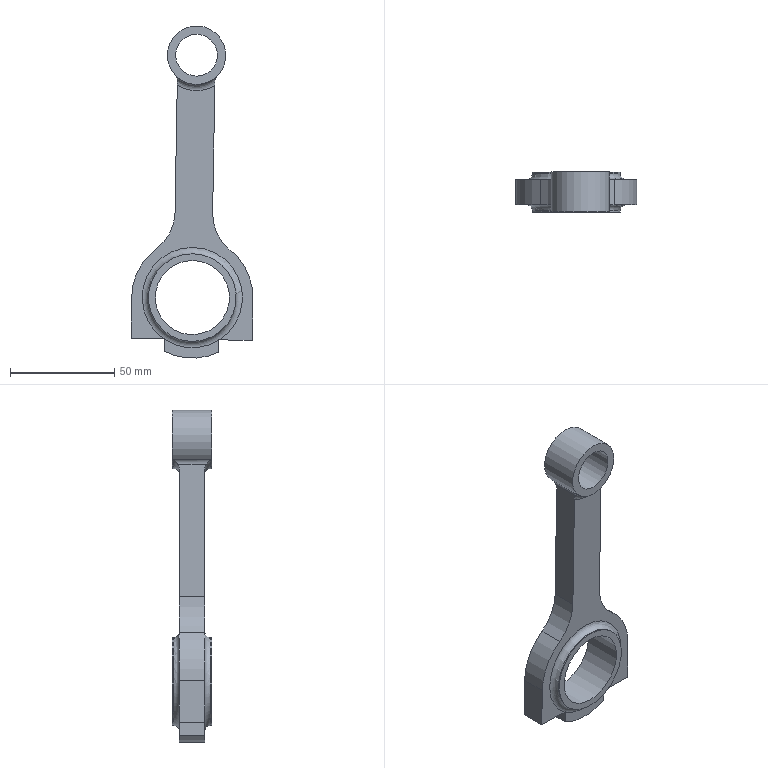Component | NX | PISTON_ROD | 1 solid | 32 faces | volume 46149 mm3 | plane 16 | cylinder 12 | torus 4 | commonest cylinder face diameters 58 x3 44 x2 42 x2 6 x2 35.5 x1 28 x1 20 x1